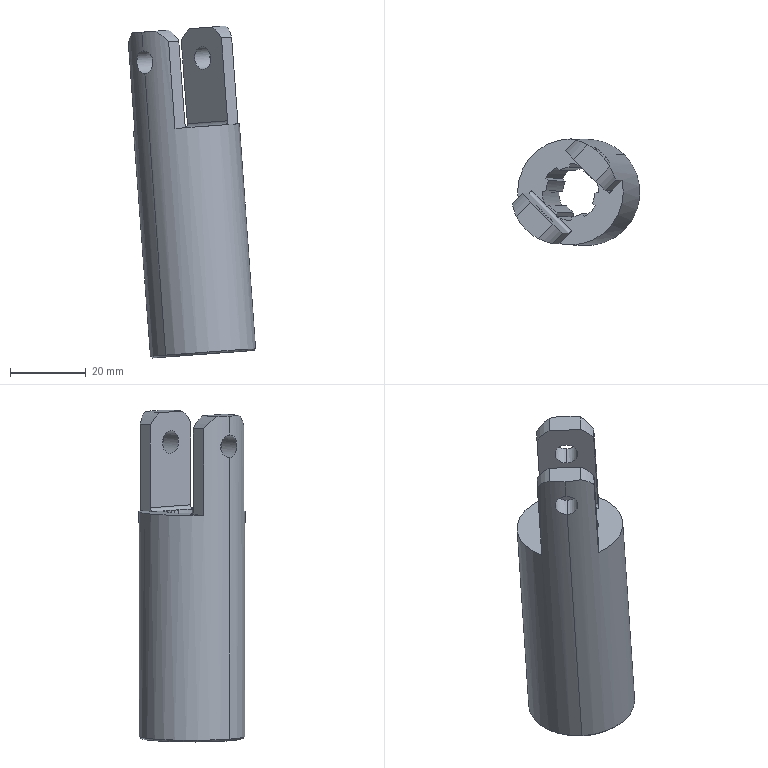Component | SolidWorks | DoubleFilmTransport-1_UniversalJointC-2 | 1 solid | 70 faces | volume 31235 mm3 | plane 37 | cylinder 25 | cone 8 | commonest cylinder face diameters 13 x7 15 x6 6 x4 18 x4 28 x2 2 x2